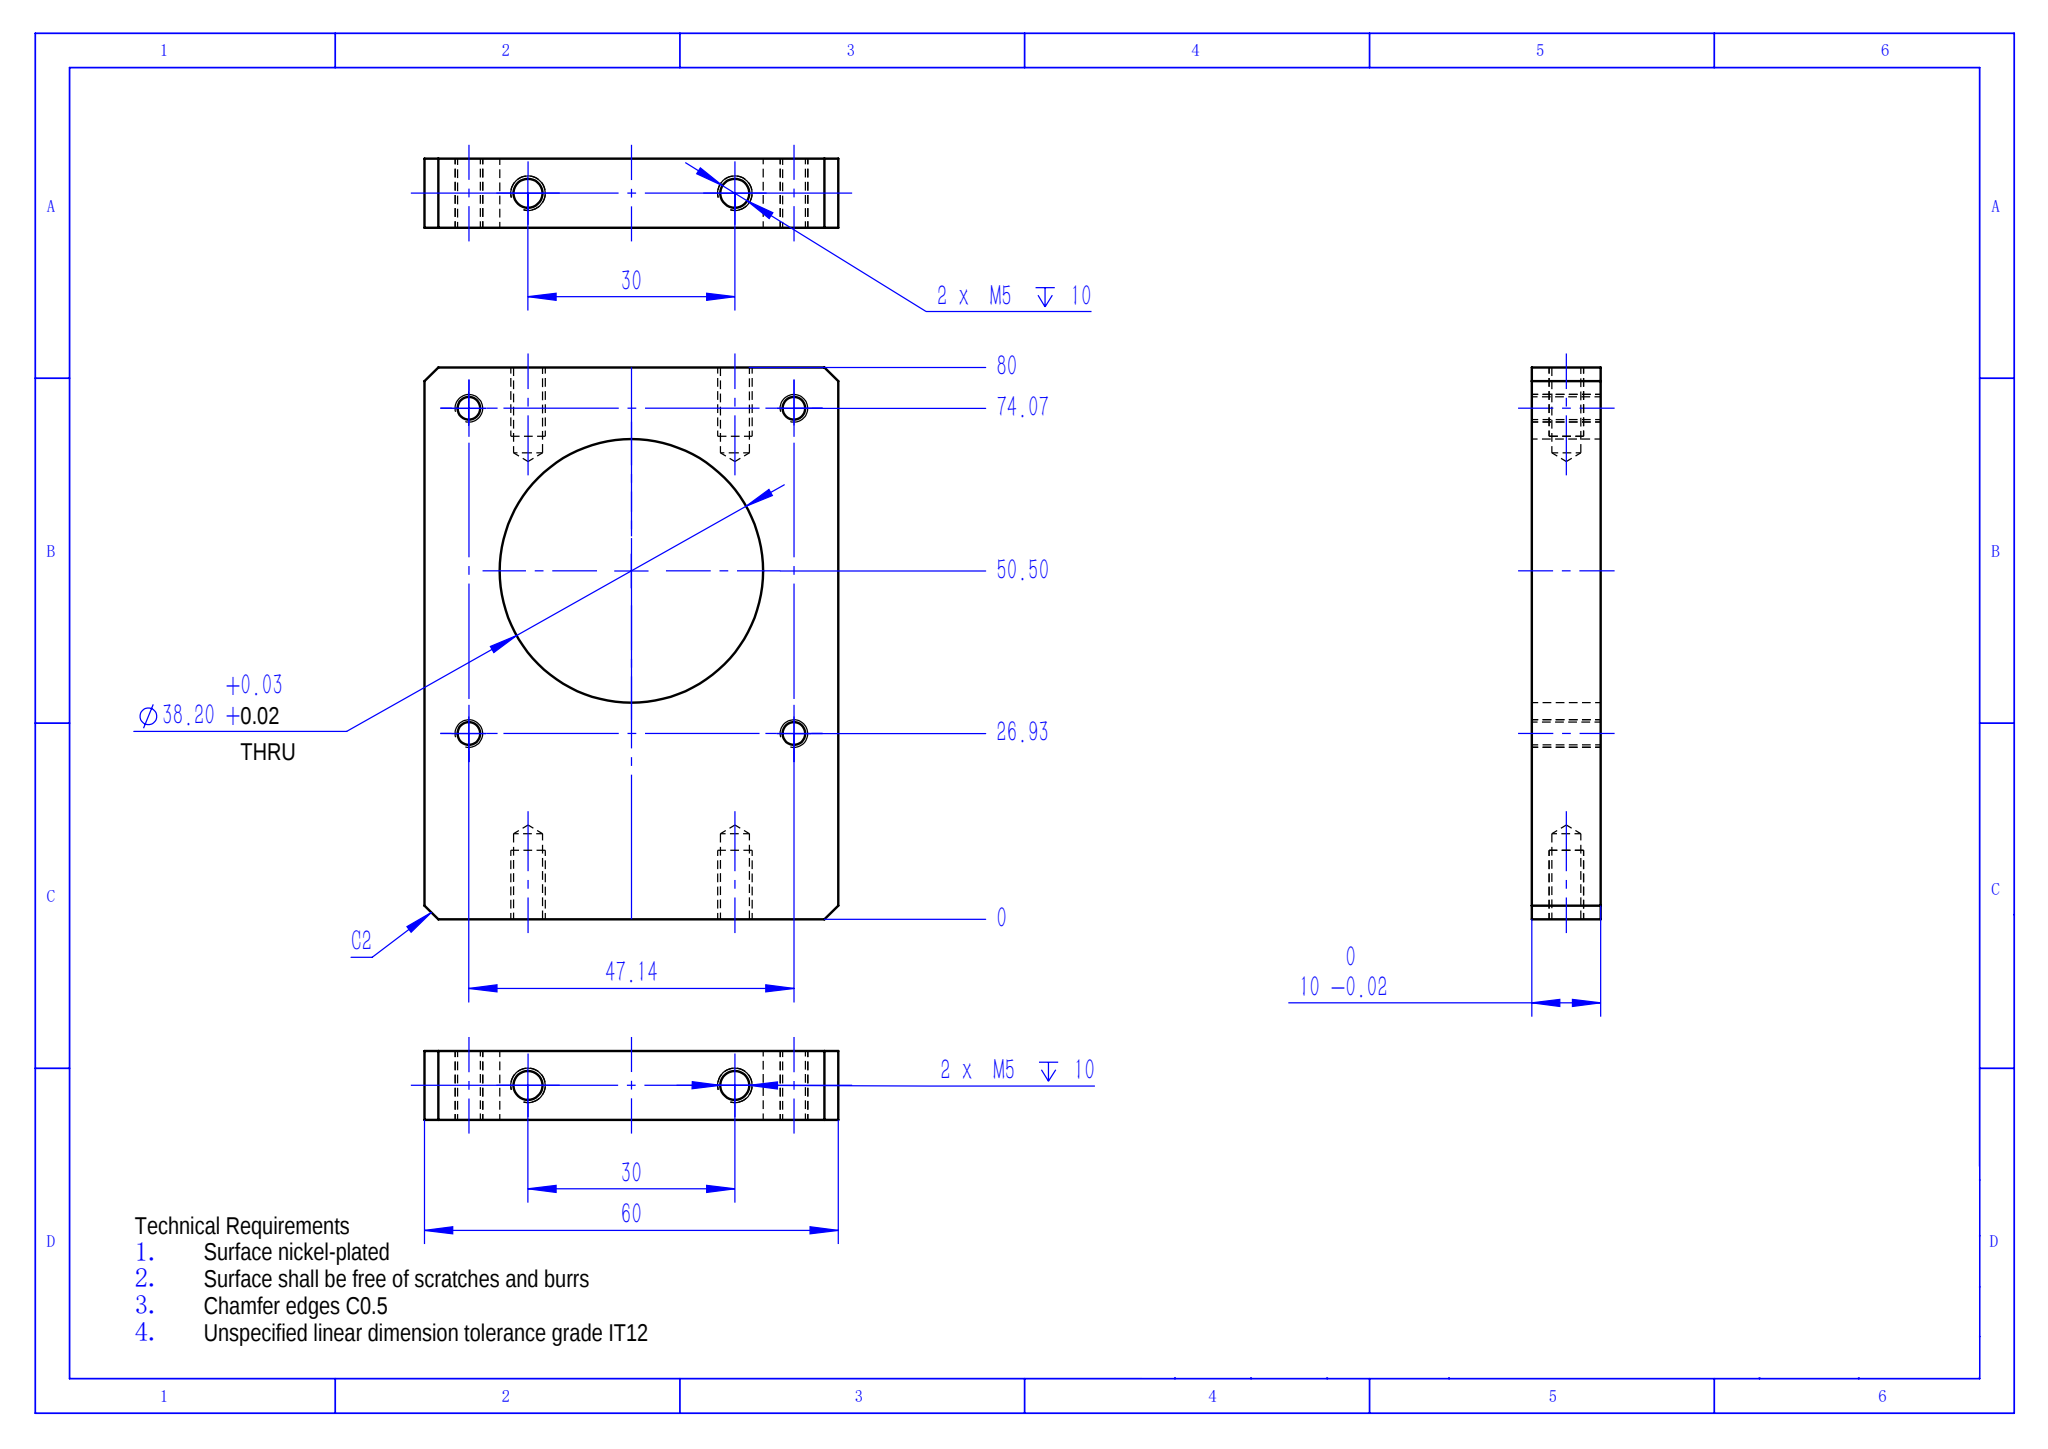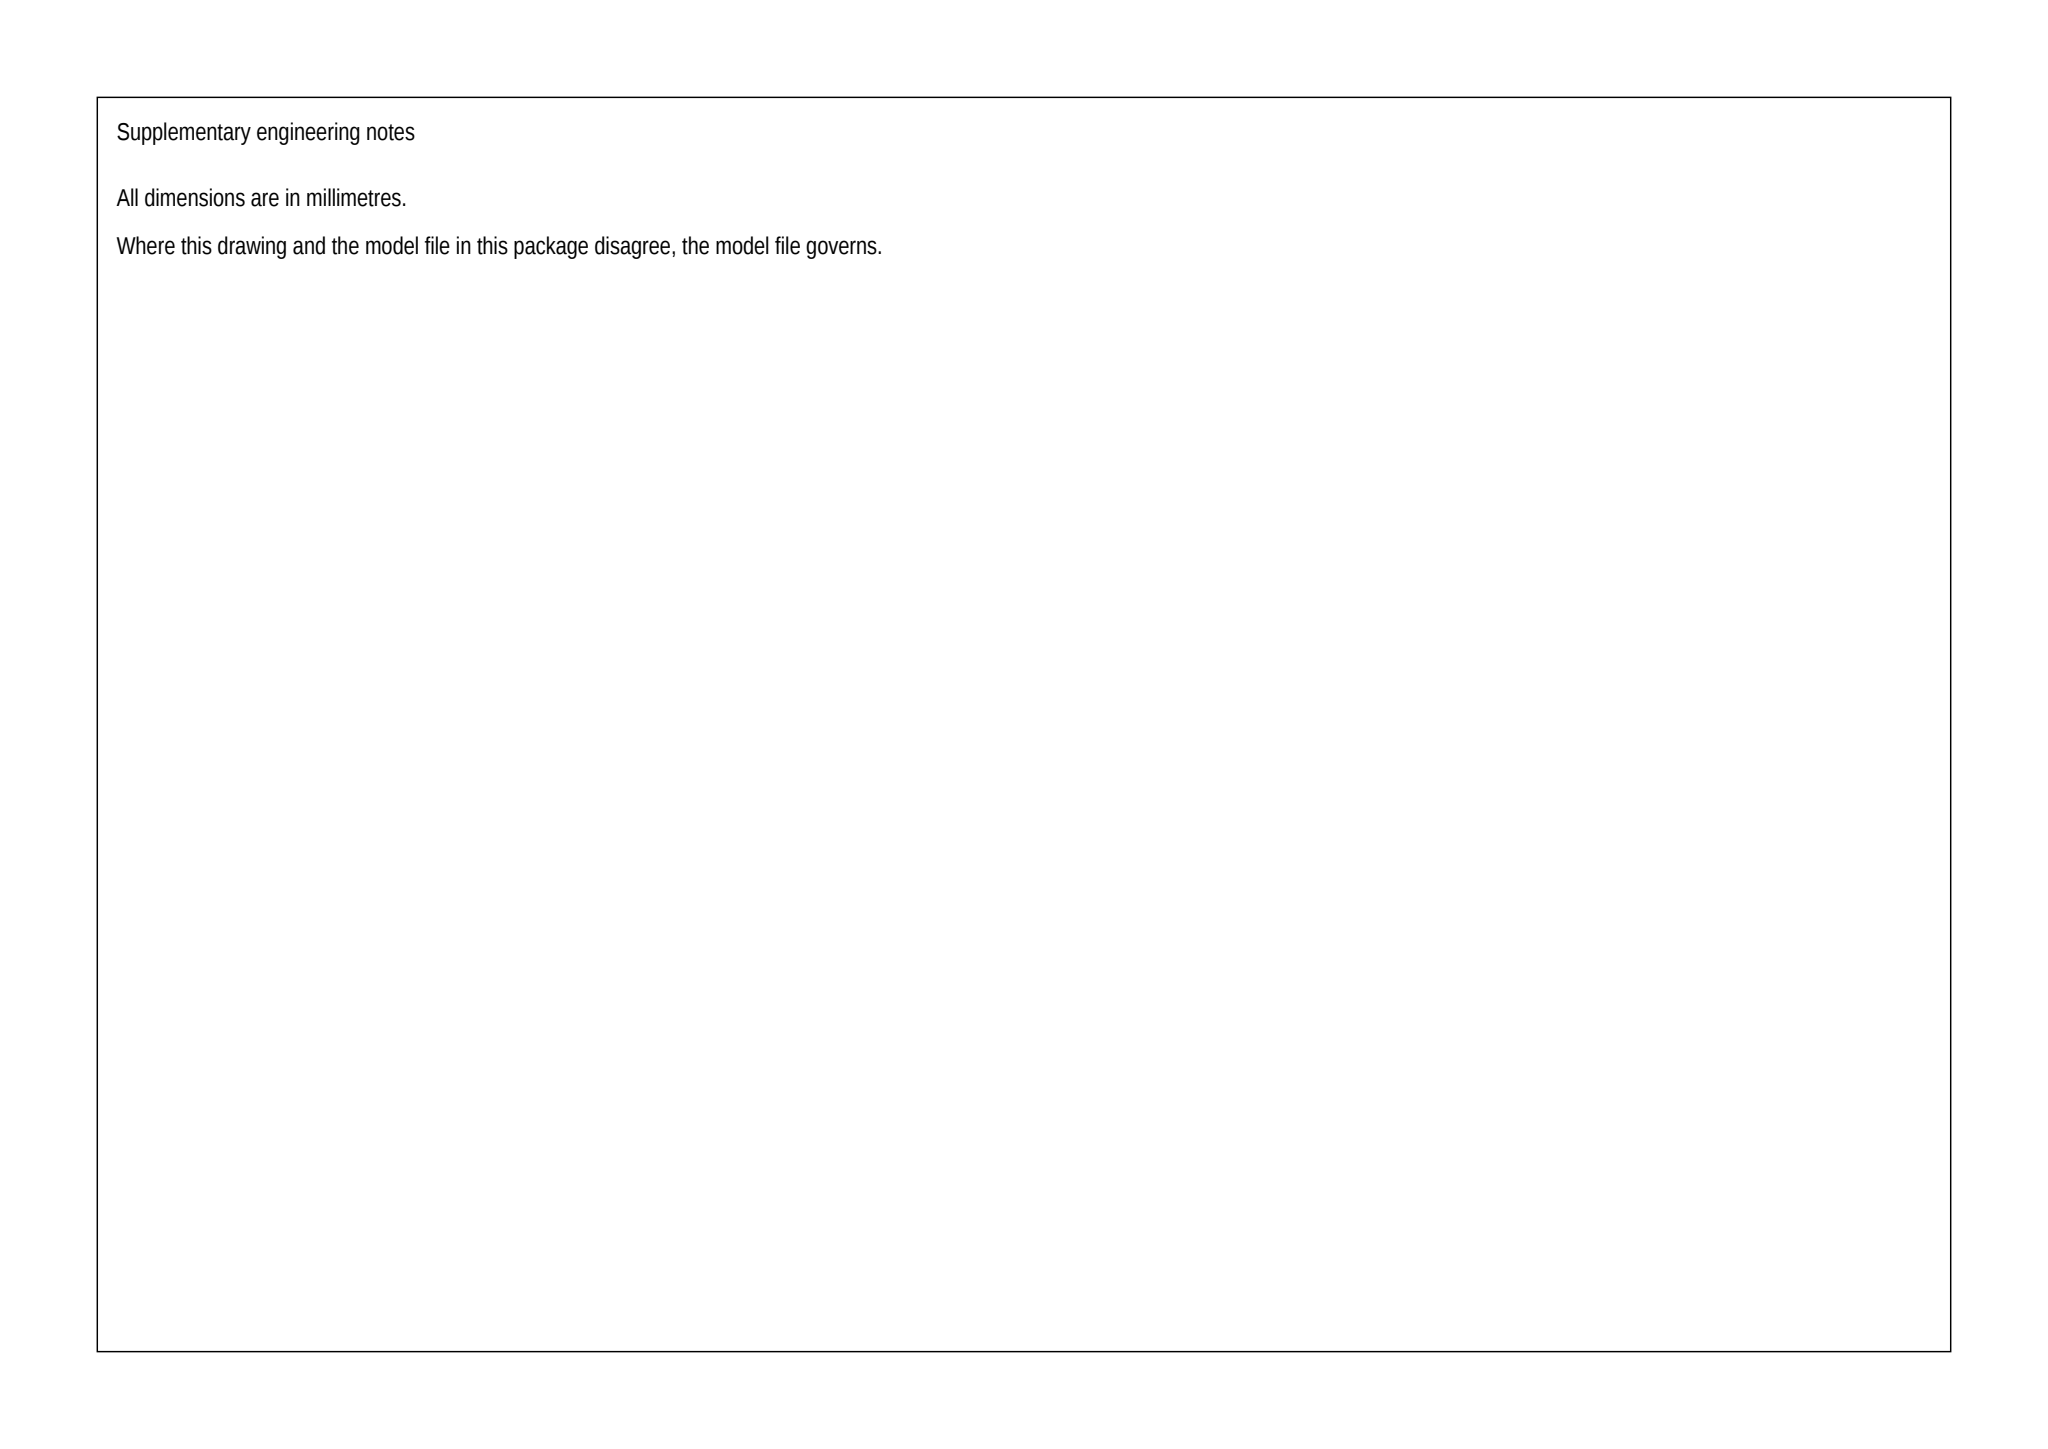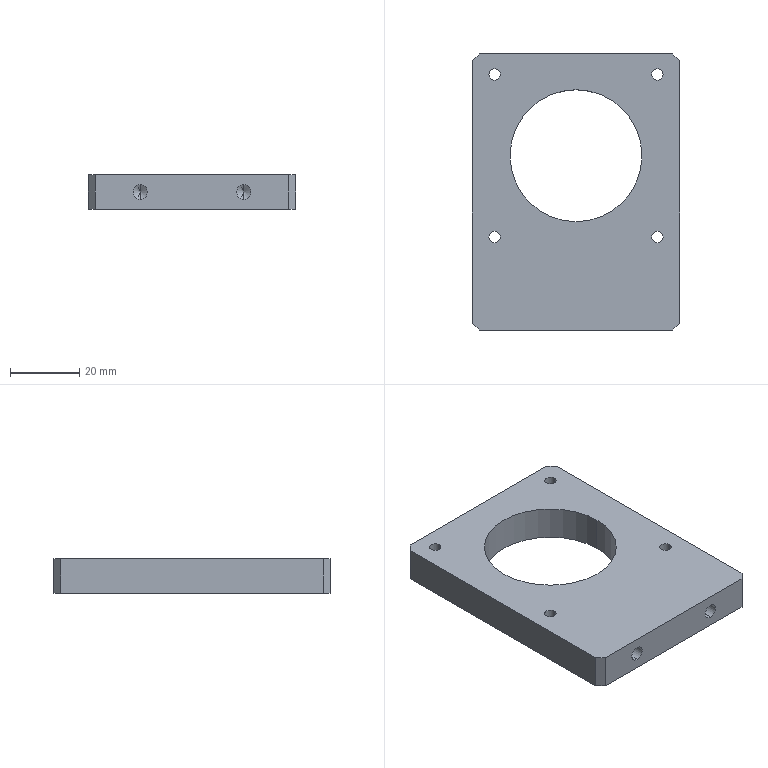Part | SolidWorks | mm | 1 solid | 36 faces | box 60 x 80 x 10 mm | volume 35407 mm3 | cylinder 18 | plane 10 | cone 8 | commonest cylinder face diameters 4.2 x8 3.3 x8 38.2 x2
build123d program:
from build123d import *

# Parameters (mm, degrees)
SKETCH1_W             = 60
SKETCH1_H             = 80
SKETCH1_R             = 19.1
BOSS_EXTRUDE1_DEPTH   = 5
M4_TAPPED_HOLE1_D     = 3.3
CHAMFER1_SIZE         = 2
M5_TAPPED_HOLE1_D     = 4.2
M5_TAPPED_HOLE1_DEPTH = 12.4
M5_TAPPED_HOLE1_TIP   = 1.262
M5_TAPPED_HOLE2_D     = 4.2
M5_TAPPED_HOLE2_DEPTH = 12.4
M5_TAPPED_HOLE2_TIP   = 1.262


with BuildPart() as part:
    # Sketch1 → Boss-Extrude1 (new, symmetric)
    with BuildSketch(Plane.XY):
        with Locations((0, -10.5)):
            Rectangle(SKETCH1_W, SKETCH1_H)
        Circle(SKETCH1_R, mode=Mode.SUBTRACT)
    extrude(amount=BOSS_EXTRUDE1_DEPTH, both=True)

    # M4 Tapped Hole1 (through all)
    with Locations(Plane(origin=(0, 0, -5), x_dir=(-1, 0, 0), z_dir=(0, 0, -1))):
        with Locations((-23.57, 23.57), (23.57, -23.57), (-23.57, -23.57), (23.57, 23.57)):
            Hole(M4_TAPPED_HOLE1_D / 2)

    # Chamfer1
    chamfer1_edges = [part.edges().sort_by_distance(p)[0] for p in [
        (-30, 29.5, 0),
        (30, 29.5, 0),
        (30, -50.5, 0),
        (-30, -50.5, 0),
    ]]
    chamfer(chamfer1_edges, length=CHAMFER1_SIZE)

    # M5 Tapped Hole1
    with Locations(Plane(origin=(0, -50.5, 0), x_dir=(-1, 0, 0), z_dir=(0, -1, 0))):
        with Locations((-15, 0), (15, 0)):
            Hole(M5_TAPPED_HOLE1_D / 2, depth=M5_TAPPED_HOLE1_DEPTH)
            with Locations((0, 0, -(M5_TAPPED_HOLE1_DEPTH + M5_TAPPED_HOLE1_TIP / 2))):  # 118° drill point
                Cone(0, M5_TAPPED_HOLE1_D / 2, M5_TAPPED_HOLE1_TIP, mode=Mode.SUBTRACT)

    # M5 Tapped Hole2
    with Locations(Plane(origin=(0, 29.5, 0), x_dir=(1, 0, 0), z_dir=(0, 1, 0))):
        with Locations((-15, 0), (15, 0)):
            Hole(M5_TAPPED_HOLE2_D / 2, depth=M5_TAPPED_HOLE2_DEPTH)
            with Locations((0, 0, -(M5_TAPPED_HOLE2_DEPTH + M5_TAPPED_HOLE2_TIP / 2))):  # 118° drill point
                Cone(0, M5_TAPPED_HOLE2_D / 2, M5_TAPPED_HOLE2_TIP, mode=Mode.SUBTRACT)


solid = part.part